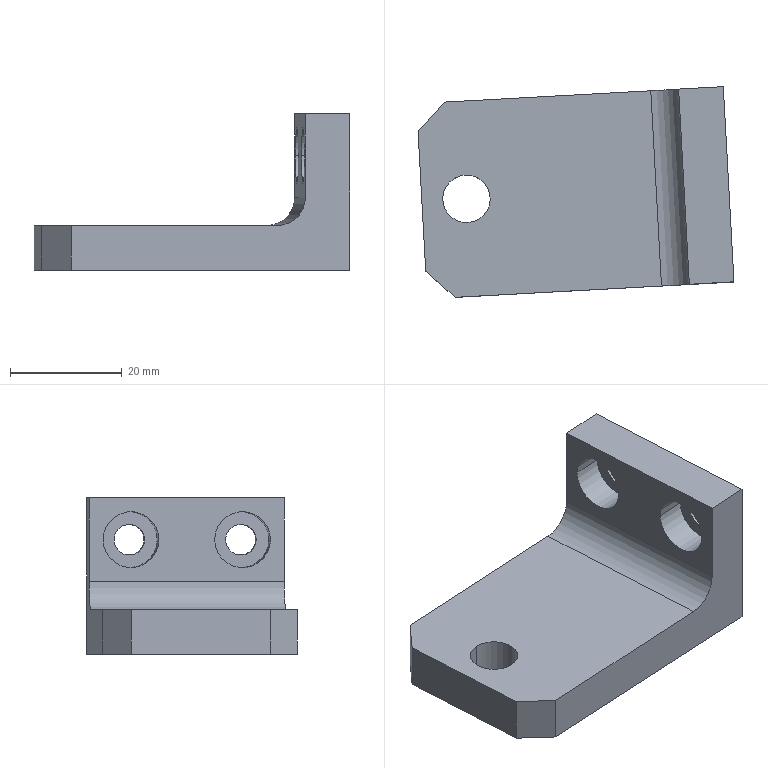Component | SolidWorks | BearingPressPartI-2 | 1 solid | 23 faces | box 56.56 x 37.68 x 28 mm | volume 19562 mm3 | plane 12 | cylinder 11 | commonest cylinder face diameters 10 x5 5.5 x4 8.5 x2
build123d program:
from build123d import *

# Parameters (mm, degrees)
BOSS_EXTRUDE1_DEPTH                             = 35
M5_HEX_SOCKET_HEAD_CAP_SCREW_CBORE1_D           = 5.5
M5_HEX_SOCKET_HEAD_CAP_SCREW_CBORE1_CBORE_D     = 10
M5_HEX_SOCKET_HEAD_CAP_SCREW_CBORE1_CBORE_DEPTH = 5.4
M10_TAPPED_HOLE1_D                              = 8.5
CHAMFER1_SIZE                                   = 5


with BuildPart() as part:
    # Sketch1 → Boss-Extrude1 (new body)
    with BuildSketch(Plane.XY):
        with BuildLine():
            Line((0, 0), (0, -55))
            Line((0, -55), (-28, -55))
            Line((-28, -55), (-28, -47))
            Line((-28, -47), (-13, -47))
            ThreePointArc((-13, -47), (-9.464, -45.536), (-8, -42))
            Line((-8, -42), (-8, 0))
            Line((-8, 0), (0, 0))
        make_face()
    extrude(amount=BOSS_EXTRUDE1_DEPTH)

    # M5 Hex Socket Head Cap Screw CBORE1 (through all)
    with Locations(Plane(origin=(0, -47, 0), x_dir=(-1, 0, 0), z_dir=(0, 1, 0))):
        with Locations((20.5, 7.5), (20.5, 27.5)):
            CounterBoreHole(M5_HEX_SOCKET_HEAD_CAP_SCREW_CBORE1_D / 2, M5_HEX_SOCKET_HEAD_CAP_SCREW_CBORE1_CBORE_D / 2, M5_HEX_SOCKET_HEAD_CAP_SCREW_CBORE1_CBORE_DEPTH)

    # M10 Tapped Hole1 (through all)
    with Locations(Plane.ZY.offset(8)):
        with Locations((17.5, -8)):
            Hole(M10_TAPPED_HOLE1_D / 2)

    # Chamfer1
    chamfer1_edges = [part.edges().sort_by_distance(p)[0] for p in [
        (-4, 0, 35),
        (-4, 0, 0),
    ]]
    chamfer(chamfer1_edges, length=CHAMFER1_SIZE)


solid = part.part

# Placed as in the assembly
solid = solid.moved(Location((341.568, 99.615, -284.318), (-90, -3.137, 90)))
STEP:
#1=COLOUR_RGB('',0.7922,0.8196,0.9333);
#2=FILL_AREA_STYLE_COLOUR('',#1);
#3=FILL_AREA_STYLE('',(#2));
#4=SURFACE_STYLE_FILL_AREA(#3);
#5=SURFACE_SIDE_STYLE('',(#4));
#6=SURFACE_STYLE_USAGE(.BOTH.,#5);
#7=PRESENTATION_STYLE_ASSIGNMENT((#6));
#8=CARTESIAN_POINT('',(13.734,4.46,-11.194));
#9=VERTEX_POINT('',#8);
#10=CARTESIAN_POINT('',(13.715,4.794,-11.194));
#11=VERTEX_POINT('',#10);
#12=CARTESIAN_POINT('',(13.724,4.627,-11.194));
#13=DIRECTION('',(0.,-0.,1.));
#14=DIRECTION('',(0.9985,0.05472,0.));
#15=AXIS2_PLACEMENT_3D('',#12,#13,#14);
#16=CIRCLE('',#15,0.1673);
#17=EDGE_CURVE('',#9,#11,#16,.T.);
#18=ORIENTED_EDGE('',*,*,#17,.F.);
#19=CARTESIAN_POINT('',(13.734,4.46,-10.879));
#20=VERTEX_POINT('',#19);
#21=CARTESIAN_POINT('',(13.734,4.46,-10.879));
#22=DIRECTION('',(0.,-0.,1.));
#23=VECTOR('',#22,39.37);
#24=LINE('',#21,#23);
#25=EDGE_CURVE('',#9,#20,#24,.T.);
#26=ORIENTED_EDGE('',*,*,#25,.T.);
#27=CARTESIAN_POINT('',(13.715,4.794,-10.879));
#28=VERTEX_POINT('',#27);
#29=CARTESIAN_POINT('',(13.724,4.627,-10.879));
#30=DIRECTION('',(0.,-0.,1.));
#31=DIRECTION('',(-0.05472,0.9985,0.));
#32=AXIS2_PLACEMENT_3D('',#29,#30,#31);
#33=CIRCLE('',#32,0.1673);
#34=EDGE_CURVE('',#20,#28,#33,.T.);
#35=ORIENTED_EDGE('',*,*,#34,.T.);
#36=CARTESIAN_POINT('',(13.715,4.794,-10.879));
#37=DIRECTION('',(0.,-0.,1.));
#38=VECTOR('',#37,39.37);
#39=LINE('',#36,#38);
#40=EDGE_CURVE('',#11,#28,#39,.T.);
#41=ORIENTED_EDGE('',*,*,#40,.F.);
#42=EDGE_LOOP('',(#18,#26,#35,#41));
#43=FACE_OUTER_BOUND('',#42,.T.);
#44=CARTESIAN_POINT('',(13.724,4.627,-10.879));
#45=DIRECTION('',(0.,-0.,1.));
#46=DIRECTION('',(-0.05472,0.9985,0.));
#47=AXIS2_PLACEMENT_3D('',#44,#45,#46);
#48=CYLINDRICAL_SURFACE('',#47,0.1673);
#49=ADVANCED_FACE('',(#43),#48,.F.);
#50=CARTESIAN_POINT('',(15.502,4.133,-10.387));
#51=VERTEX_POINT('',#50);
#52=CARTESIAN_POINT('',(15.481,4.526,-10.387));
#53=VERTEX_POINT('',#52);
#54=CARTESIAN_POINT('',(15.491,4.33,-10.387));
#55=DIRECTION('',(-0.9985,-0.05472,0.));
#56=DIRECTION('',(-0.05472,0.9985,0.));
#57=AXIS2_PLACEMENT_3D('',#54,#55,#56);
#58=CIRCLE('',#57,0.1969);
#59=EDGE_CURVE('',#51,#53,#58,.T.);
#60=ORIENTED_EDGE('',*,*,#59,.F.);
#61=CARTESIAN_POINT('',(15.29,4.121,-10.387));
#62=VERTEX_POINT('',#61);
#63=CARTESIAN_POINT('',(15.29,4.121,-10.387));
#64=DIRECTION('',(-0.9985,-0.05472,0.));
#65=VECTOR('',#64,39.37);
#66=LINE('',#63,#65);
#67=EDGE_CURVE('',#51,#62,#66,.T.);
#68=ORIENTED_EDGE('',*,*,#67,.T.);
#69=CARTESIAN_POINT('',(15.268,4.515,-10.387));
#70=VERTEX_POINT('',#69);
#71=CARTESIAN_POINT('',(15.279,4.318,-10.387));
#72=DIRECTION('',(-0.9985,-0.05472,0.));
#73=DIRECTION('',(-0.05472,0.9985,0.));
#74=AXIS2_PLACEMENT_3D('',#71,#72,#73);
#75=CIRCLE('',#74,0.1969);
#76=EDGE_CURVE('',#62,#70,#75,.T.);
#77=ORIENTED_EDGE('',*,*,#76,.T.);
#78=CARTESIAN_POINT('',(15.268,4.515,-10.387));
#79=DIRECTION('',(-0.9985,-0.05472,0.));
#80=VECTOR('',#79,39.37);
#81=LINE('',#78,#80);
#82=EDGE_CURVE('',#53,#70,#81,.T.);
#83=ORIENTED_EDGE('',*,*,#82,.F.);
#84=EDGE_LOOP('',(#60,#68,#77,#83));
#85=FACE_OUTER_BOUND('',#84,.T.);
#86=CARTESIAN_POINT('',(15.279,4.318,-10.387));
#87=DIRECTION('',(-0.9985,-0.05472,0.));
#88=DIRECTION('',(-0.05472,0.9985,0.));
#89=AXIS2_PLACEMENT_3D('',#86,#87,#88);
#90=CYLINDRICAL_SURFACE('',#89,0.1969);
#91=ADVANCED_FACE('',(#85),#90,.F.);
#92=CARTESIAN_POINT('',(15.599,4.227,-10.387));
#93=VERTEX_POINT('',#92);
#94=CARTESIAN_POINT('',(15.588,4.443,-10.387));
#95=VERTEX_POINT('',#94);
#96=CARTESIAN_POINT('',(15.594,4.335,-10.387));
#97=DIRECTION('',(-0.9985,-0.05472,0.));
#98=DIRECTION('',(0.,0.,1.));
#99=AXIS2_PLACEMENT_3D('',#96,#97,#98);
#100=CIRCLE('',#99,0.1083);
#101=EDGE_CURVE('',#93,#95,#100,.T.);
#102=ORIENTED_EDGE('',*,*,#101,.F.);
#103=CARTESIAN_POINT('',(15.497,4.221,-10.387));
#104=VERTEX_POINT('',#103);
#105=CARTESIAN_POINT('',(15.285,4.21,-10.387));
#106=DIRECTION('',(-0.9985,-0.05472,0.));
#107=VECTOR('',#106,39.37);
#108=LINE('',#105,#107);
#109=EDGE_CURVE('',#93,#104,#108,.T.);
#110=ORIENTED_EDGE('',*,*,#109,.T.);
#111=CARTESIAN_POINT('',(15.485,4.438,-10.387));
#112=VERTEX_POINT('',#111);
#113=CARTESIAN_POINT('',(15.491,4.33,-10.387));
#114=DIRECTION('',(-0.9985,-0.05472,0.));
#115=DIRECTION('',(-0.05472,0.9985,0.));
#116=AXIS2_PLACEMENT_3D('',#113,#114,#115);
#117=CIRCLE('',#116,0.1083);
#118=EDGE_CURVE('',#104,#112,#117,.T.);
#119=ORIENTED_EDGE('',*,*,#118,.T.);
#120=CARTESIAN_POINT('',(15.273,4.426,-10.387));
#121=DIRECTION('',(-0.9985,-0.05472,0.));
#122=VECTOR('',#121,39.37);
#123=LINE('',#120,#122);
#124=EDGE_CURVE('',#95,#112,#123,.T.);
#125=ORIENTED_EDGE('',*,*,#124,.F.);
#126=EDGE_LOOP('',(#102,#110,#119,#125));
#127=FACE_OUTER_BOUND('',#126,.T.);
#128=CARTESIAN_POINT('',(15.279,4.318,-10.387));
#129=DIRECTION('',(-0.9985,-0.05472,0.));
#130=DIRECTION('',(-0.05472,0.9985,0.));
#131=AXIS2_PLACEMENT_3D('',#128,#129,#130);
#132=CYLINDRICAL_SURFACE('',#131,0.1083);
#133=ADVANCED_FACE('',(#127),#132,.F.);
#134=CARTESIAN_POINT('',(15.459,4.919,-10.387));
#135=VERTEX_POINT('',#134);
#136=CARTESIAN_POINT('',(15.437,5.312,-10.387));
#137=VERTEX_POINT('',#136);
#138=CARTESIAN_POINT('',(15.448,5.116,-10.387));
#139=DIRECTION('',(-0.9985,-0.05472,0.));
#140=DIRECTION('',(-0.05472,0.9985,0.));
#141=AXIS2_PLACEMENT_3D('',#138,#139,#140);
#142=CIRCLE('',#141,0.1969);
#143=EDGE_CURVE('',#135,#137,#142,.T.);
#144=ORIENTED_EDGE('',*,*,#143,.F.);
#145=CARTESIAN_POINT('',(15.247,4.908,-10.387));
#146=VERTEX_POINT('',#145);
#147=CARTESIAN_POINT('',(15.247,4.908,-10.387));
#148=DIRECTION('',(-0.9985,-0.05472,0.));
#149=VECTOR('',#148,39.37);
#150=LINE('',#147,#149);
#151=EDGE_CURVE('',#135,#146,#150,.T.);
#152=ORIENTED_EDGE('',*,*,#151,.T.);
#153=CARTESIAN_POINT('',(15.225,5.301,-10.387));
#154=VERTEX_POINT('',#153);
#155=CARTESIAN_POINT('',(15.236,5.104,-10.387));
#156=DIRECTION('',(-0.9985,-0.05472,0.));
#157=DIRECTION('',(-0.05472,0.9985,0.));
#158=AXIS2_PLACEMENT_3D('',#155,#156,#157);
#159=CIRCLE('',#158,0.1969);
#160=EDGE_CURVE('',#146,#154,#159,.T.);
#161=ORIENTED_EDGE('',*,*,#160,.T.);
#162=CARTESIAN_POINT('',(15.225,5.301,-10.387));
#163=DIRECTION('',(-0.9985,-0.05472,0.));
#164=VECTOR('',#163,39.37);
#165=LINE('',#162,#164);
#166=EDGE_CURVE('',#137,#154,#165,.T.);
#167=ORIENTED_EDGE('',*,*,#166,.F.);
#168=EDGE_LOOP('',(#144,#152,#161,#167));
#169=FACE_OUTER_BOUND('',#168,.T.);
#170=CARTESIAN_POINT('',(15.236,5.104,-10.387));
#171=DIRECTION('',(-0.9985,-0.05472,0.));
#172=DIRECTION('',(-0.05472,0.9985,0.));
#173=AXIS2_PLACEMENT_3D('',#170,#171,#172);
#174=CYLINDRICAL_SURFACE('',#173,0.1969);
#175=ADVANCED_FACE('',(#169),#174,.F.);
#176=CARTESIAN_POINT('',(15.556,5.013,-10.387));
#177=VERTEX_POINT('',#176);
#178=CARTESIAN_POINT('',(15.545,5.23,-10.387));
#179=VERTEX_POINT('',#178);
#180=CARTESIAN_POINT('',(15.55,5.121,-10.387));
#181=DIRECTION('',(-0.9985,-0.05472,0.));
#182=DIRECTION('',(0.,0.,1.));
#183=AXIS2_PLACEMENT_3D('',#180,#181,#182);
#184=CIRCLE('',#183,0.1083);
#185=EDGE_CURVE('',#177,#179,#184,.T.);
#186=ORIENTED_EDGE('',*,*,#185,.F.);
#187=CARTESIAN_POINT('',(15.454,5.008,-10.387));
#188=VERTEX_POINT('',#187);
#189=CARTESIAN_POINT('',(15.242,4.996,-10.387));
#190=DIRECTION('',(-0.9985,-0.05472,0.));
#191=VECTOR('',#190,39.37);
#192=LINE('',#189,#191);
#193=EDGE_CURVE('',#177,#188,#192,.T.);
#194=ORIENTED_EDGE('',*,*,#193,.T.);
#195=CARTESIAN_POINT('',(15.442,5.224,-10.387));
#196=VERTEX_POINT('',#195);
#197=CARTESIAN_POINT('',(15.448,5.116,-10.387));
#198=DIRECTION('',(-0.9985,-0.05472,0.));
#199=DIRECTION('',(-0.05472,0.9985,0.));
#200=AXIS2_PLACEMENT_3D('',#197,#198,#199);
#201=CIRCLE('',#200,0.1083);
#202=EDGE_CURVE('',#188,#196,#201,.T.);
#203=ORIENTED_EDGE('',*,*,#202,.T.);
#204=CARTESIAN_POINT('',(15.23,5.212,-10.387));
#205=DIRECTION('',(-0.9985,-0.05472,0.));
#206=VECTOR('',#205,39.37);
#207=LINE('',#204,#206);
#208=EDGE_CURVE('',#179,#196,#207,.T.);
#209=ORIENTED_EDGE('',*,*,#208,.F.);
#210=EDGE_LOOP('',(#186,#194,#203,#209));
#211=FACE_OUTER_BOUND('',#210,.T.);
#212=CARTESIAN_POINT('',(15.236,5.104,-10.387));
#213=DIRECTION('',(-0.9985,-0.05472,0.));
#214=DIRECTION('',(-0.05472,0.9985,0.));
#215=AXIS2_PLACEMENT_3D('',#212,#213,#214);
#216=CYLINDRICAL_SURFACE('',#215,0.1083);
#217=ADVANCED_FACE('',(#211),#216,.F.);
#218=CARTESIAN_POINT('',(15.295,4.023,-10.682));
#219=VERTEX_POINT('',#218);
#220=CARTESIAN_POINT('',(15.295,4.023,-10.091));
#221=VERTEX_POINT('',#220);
#222=CARTESIAN_POINT('',(15.295,4.023,-10.091));
#223=DIRECTION('',(0.,-0.,1.));
#224=VECTOR('',#223,39.37);
#225=LINE('',#222,#224);
#226=EDGE_CURVE('',#219,#221,#225,.T.);
#227=ORIENTED_EDGE('',*,*,#226,.T.);
#228=CARTESIAN_POINT('',(15.22,5.399,-10.091));
#229=VERTEX_POINT('',#228);
#230=CARTESIAN_POINT('',(15.22,5.399,-10.091));
#231=DIRECTION('',(0.05472,-0.9985,-0.));
#232=VECTOR('',#231,39.37);
#233=LINE('',#230,#232);
#234=EDGE_CURVE('',#229,#221,#233,.T.);
#235=ORIENTED_EDGE('',*,*,#234,.F.);
#236=CARTESIAN_POINT('',(15.22,5.399,-10.682));
#237=VERTEX_POINT('',#236);
#238=CARTESIAN_POINT('',(15.22,5.399,-10.091));
#239=DIRECTION('',(0.,-0.,1.));
#240=VECTOR('',#239,39.37);
#241=LINE('',#238,#240);
#242=EDGE_CURVE('',#237,#229,#241,.T.);
#243=ORIENTED_EDGE('',*,*,#242,.F.);
#244=CARTESIAN_POINT('',(15.22,5.399,-10.682));
#245=DIRECTION('',(0.05472,-0.9985,-0.));
#246=VECTOR('',#245,39.37);
#247=LINE('',#244,#246);
#248=EDGE_CURVE('',#237,#219,#247,.T.);
#249=ORIENTED_EDGE('',*,*,#248,.T.);
#250=EDGE_LOOP('',(#227,#235,#243,#249));
#251=FACE_OUTER_BOUND('',#250,.T.);
#252=CARTESIAN_POINT('',(15.236,5.104,-10.387));
#253=DIRECTION('',(-0.9985,-0.05472,0.));
#254=DIRECTION('',(-0.05472,0.9985,0.));
#255=AXIS2_PLACEMENT_3D('',#252,#253,#254);
#256=CIRCLE('',#255,0.1969);
#257=EDGE_CURVE('',#154,#146,#256,.T.);
#258=ORIENTED_EDGE('',*,*,#257,.F.);
#259=ORIENTED_EDGE('',*,*,#160,.F.);
#260=EDGE_LOOP('',(#258,#259));
#261=FACE_BOUND('',#260,.T.);
#262=CARTESIAN_POINT('',(15.279,4.318,-10.387));
#263=DIRECTION('',(-0.9985,-0.05472,0.));
#264=DIRECTION('',(-0.05472,0.9985,0.));
#265=AXIS2_PLACEMENT_3D('',#262,#263,#264);
#266=CIRCLE('',#265,0.1969);
#267=EDGE_CURVE('',#70,#62,#266,.T.);
#268=ORIENTED_EDGE('',*,*,#267,.F.);
#269=ORIENTED_EDGE('',*,*,#76,.F.);
#270=EDGE_LOOP('',(#268,#269));
#271=FACE_BOUND('',#270,.T.);
#272=CARTESIAN_POINT('',(15.22,5.399,-10.091));
#273=DIRECTION('',(0.9985,0.05472,-0.));
#274=DIRECTION('',(0.05472,-0.9985,-0.));
#275=AXIS2_PLACEMENT_3D('',#272,#273,#274);
#276=PLANE('',#275);
#277=ADVANCED_FACE('',(#251,#261,#271),#276,.F.);
#278=CARTESIAN_POINT('',(13.383,5.101,-11.194));
#279=VERTEX_POINT('',#278);
#280=CARTESIAN_POINT('',(13.437,4.118,-11.194));
#281=VERTEX_POINT('',#280);
#282=CARTESIAN_POINT('',(13.372,5.298,-11.194));
#283=DIRECTION('',(0.05472,-0.9985,-0.));
#284=VECTOR('',#283,39.37);
#285=LINE('',#282,#284);
#286=EDGE_CURVE('',#279,#281,#285,.T.);
#287=ORIENTED_EDGE('',*,*,#286,.T.);
#288=CARTESIAN_POINT('',(13.437,4.118,-10.879));
#289=VERTEX_POINT('',#288);
#290=CARTESIAN_POINT('',(13.437,4.118,-10.879));
#291=DIRECTION('',(0.,-0.,1.));
#292=VECTOR('',#291,39.37);
#293=LINE('',#290,#292);
#294=EDGE_CURVE('',#281,#289,#293,.T.);
#295=ORIENTED_EDGE('',*,*,#294,.T.);
#296=CARTESIAN_POINT('',(13.383,5.101,-10.879));
#297=VERTEX_POINT('',#296);
#298=CARTESIAN_POINT('',(13.372,5.298,-10.879));
#299=DIRECTION('',(0.05472,-0.9985,-0.));
#300=VECTOR('',#299,39.37);
#301=LINE('',#298,#300);
#302=EDGE_CURVE('',#297,#289,#301,.T.);
#303=ORIENTED_EDGE('',*,*,#302,.F.);
#304=CARTESIAN_POINT('',(13.383,5.101,-10.879));
#305=DIRECTION('',(-0.,0.,-1.));
#306=VECTOR('',#305,39.37);
#307=LINE('',#304,#306);
#308=EDGE_CURVE('',#297,#279,#307,.T.);
#309=ORIENTED_EDGE('',*,*,#308,.T.);
#310=EDGE_LOOP('',(#287,#295,#303,#309));
#311=FACE_OUTER_BOUND('',#310,.T.);
#312=CARTESIAN_POINT('',(13.372,5.298,-10.879));
#313=DIRECTION('',(0.9985,0.05472,-0.));
#314=DIRECTION('',(0.05472,-0.9985,-0.));
#315=AXIS2_PLACEMENT_3D('',#312,#313,#314);
#316=PLANE('',#315);
#317=ADVANCED_FACE('',(#311),#316,.F.);
#318=CARTESIAN_POINT('',(13.724,4.627,-10.879));
#319=DIRECTION('',(0.,-0.,1.));
#320=DIRECTION('',(-0.05472,0.9985,0.));
#321=AXIS2_PLACEMENT_3D('',#318,#319,#320);
#322=CIRCLE('',#321,0.1673);
#323=EDGE_CURVE('',#28,#20,#322,.T.);
#324=ORIENTED_EDGE('',*,*,#323,.F.);
#325=ORIENTED_EDGE('',*,*,#34,.F.);
#326=EDGE_LOOP('',(#324,#325));
#327=FACE_BOUND('',#326,.T.);
#328=ORIENTED_EDGE('',*,*,#302,.T.);
#329=CARTESIAN_POINT('',(13.644,3.933,-10.879));
#330=VERTEX_POINT('',#329);
#331=CARTESIAN_POINT('',(13.437,4.118,-10.879));
#332=DIRECTION('',(0.7447,-0.6674,-0.));
#333=VECTOR('',#332,39.37);
#334=LINE('',#331,#333);
#335=EDGE_CURVE('',#289,#330,#334,.T.);
#336=ORIENTED_EDGE('',*,*,#335,.T.);
#337=CARTESIAN_POINT('',(15.099,4.012,-10.879));
#338=VERTEX_POINT('',#337);
#339=CARTESIAN_POINT('',(15.099,4.012,-10.879));
#340=DIRECTION('',(0.9985,0.05472,-0.));
#341=VECTOR('',#340,39.37);
#342=LINE('',#339,#341);
#343=EDGE_CURVE('',#330,#338,#342,.T.);
#344=ORIENTED_EDGE('',*,*,#343,.T.);
#345=CARTESIAN_POINT('',(15.023,5.388,-10.879));
#346=VERTEX_POINT('',#345);
#347=CARTESIAN_POINT('',(15.023,5.388,-10.879));
#348=DIRECTION('',(0.05472,-0.9985,-0.));
#349=VECTOR('',#348,39.37);
#350=LINE('',#347,#349);
#351=EDGE_CURVE('',#346,#338,#350,.T.);
#352=ORIENTED_EDGE('',*,*,#351,.F.);
#353=CARTESIAN_POINT('',(13.569,5.309,-10.879));
#354=VERTEX_POINT('',#353);
#355=CARTESIAN_POINT('',(15.023,5.388,-10.879));
#356=DIRECTION('',(0.9985,0.05472,-0.));
#357=VECTOR('',#356,39.37);
#358=LINE('',#355,#357);
#359=EDGE_CURVE('',#354,#346,#358,.T.);
#360=ORIENTED_EDGE('',*,*,#359,.F.);
#361=CARTESIAN_POINT('',(13.569,5.309,-10.879));
#362=DIRECTION('',(-0.6674,-0.7447,-0.));
#363=VECTOR('',#362,39.37);
#364=LINE('',#361,#363);
#365=EDGE_CURVE('',#354,#297,#364,.T.);
#366=ORIENTED_EDGE('',*,*,#365,.T.);
#367=EDGE_LOOP('',(#328,#336,#344,#352,#360,#366));
#368=FACE_OUTER_BOUND('',#367,.T.);
#369=CARTESIAN_POINT('',(15.023,5.388,-10.879));
#370=DIRECTION('',(-0.,0.,-1.));
#371=DIRECTION('',(0.05472,-0.9985,-0.));
#372=AXIS2_PLACEMENT_3D('',#369,#370,#371);
#373=PLANE('',#372);
#374=ADVANCED_FACE('',(#327,#368),#373,.F.);
#375=CARTESIAN_POINT('',(15.099,4.012,-10.682));
#376=DIRECTION('',(0.05472,-0.9985,-0.));
#377=DIRECTION('',(0.,0.,1.));
#378=AXIS2_PLACEMENT_3D('',#375,#376,#377);
#379=CIRCLE('',#378,0.1969);
#380=EDGE_CURVE('',#338,#219,#379,.T.);
#381=ORIENTED_EDGE('',*,*,#380,.T.);
#382=ORIENTED_EDGE('',*,*,#248,.F.);
#383=CARTESIAN_POINT('',(15.023,5.388,-10.682));
#384=DIRECTION('',(0.05472,-0.9985,-0.));
#385=DIRECTION('',(0.,0.,1.));
#386=AXIS2_PLACEMENT_3D('',#383,#384,#385);
#387=CIRCLE('',#386,0.1969);
#388=EDGE_CURVE('',#346,#237,#387,.T.);
#389=ORIENTED_EDGE('',*,*,#388,.F.);
#390=ORIENTED_EDGE('',*,*,#351,.T.);
#391=EDGE_LOOP('',(#381,#382,#389,#390));
#392=FACE_OUTER_BOUND('',#391,.T.);
#393=CARTESIAN_POINT('',(15.023,5.388,-10.682));
#394=DIRECTION('',(0.05472,-0.9985,-0.));
#395=DIRECTION('',(0.,0.,1.));
#396=AXIS2_PLACEMENT_3D('',#393,#394,#395);
#397=CYLINDRICAL_SURFACE('',#396,0.1969);
#398=ADVANCED_FACE('',(#392),#397,.F.);
#399=CARTESIAN_POINT('',(15.61,4.04,-10.091));
#400=VERTEX_POINT('',#399);
#401=CARTESIAN_POINT('',(15.61,4.04,-10.091));
#402=DIRECTION('',(0.9985,0.05472,-0.));
#403=VECTOR('',#402,39.37);
#404=LINE('',#401,#403);
#405=EDGE_CURVE('',#221,#400,#404,.T.);
#406=ORIENTED_EDGE('',*,*,#405,.T.);
#407=CARTESIAN_POINT('',(15.534,5.416,-10.091));
#408=VERTEX_POINT('',#407);
#409=CARTESIAN_POINT('',(15.534,5.416,-10.091));
#410=DIRECTION('',(0.05472,-0.9985,-0.));
#411=VECTOR('',#410,39.37);
#412=LINE('',#409,#411);
#413=EDGE_CURVE('',#408,#400,#412,.T.);
#414=ORIENTED_EDGE('',*,*,#413,.F.);
#415=CARTESIAN_POINT('',(15.534,5.416,-10.091));
#416=DIRECTION('',(0.9985,0.05472,-0.));
#417=VECTOR('',#416,39.37);
#418=LINE('',#415,#417);
#419=EDGE_CURVE('',#229,#408,#418,.T.);
#420=ORIENTED_EDGE('',*,*,#419,.F.);
#421=ORIENTED_EDGE('',*,*,#234,.T.);
#422=EDGE_LOOP('',(#406,#414,#420,#421));
#423=FACE_OUTER_BOUND('',#422,.T.);
#424=CARTESIAN_POINT('',(15.534,5.416,-10.091));
#425=DIRECTION('',(-0.,0.,-1.));
#426=DIRECTION('',(0.05472,-0.9985,-0.));
#427=AXIS2_PLACEMENT_3D('',#424,#425,#426);
#428=PLANE('',#427);
#429=ADVANCED_FACE('',(#423),#428,.F.);
#430=CARTESIAN_POINT('',(15.594,4.335,-10.387));
#431=DIRECTION('',(-0.9985,-0.05472,0.));
#432=DIRECTION('',(0.,0.,1.));
#433=AXIS2_PLACEMENT_3D('',#430,#431,#432);
#434=CIRCLE('',#433,0.1083);
#435=EDGE_CURVE('',#95,#93,#434,.T.);
#436=ORIENTED_EDGE('',*,*,#435,.T.);
#437=ORIENTED_EDGE('',*,*,#101,.T.);
#438=EDGE_LOOP('',(#436,#437));
#439=FACE_BOUND('',#438,.T.);
#440=CARTESIAN_POINT('',(15.55,5.121,-10.387));
#441=DIRECTION('',(-0.9985,-0.05472,0.));
#442=DIRECTION('',(0.,0.,1.));
#443=AXIS2_PLACEMENT_3D('',#440,#441,#442);
#444=CIRCLE('',#443,0.1083);
#445=EDGE_CURVE('',#179,#177,#444,.T.);
#446=ORIENTED_EDGE('',*,*,#445,.T.);
#447=ORIENTED_EDGE('',*,*,#185,.T.);
#448=EDGE_LOOP('',(#446,#447));
#449=FACE_BOUND('',#448,.T.);
#450=CARTESIAN_POINT('',(15.61,4.04,-11.194));
#451=VERTEX_POINT('',#450);
#452=CARTESIAN_POINT('',(15.61,4.04,-11.194));
#453=DIRECTION('',(-0.,0.,-1.));
#454=VECTOR('',#453,39.37);
#455=LINE('',#452,#454);
#456=EDGE_CURVE('',#400,#451,#455,.T.);
#457=ORIENTED_EDGE('',*,*,#456,.T.);
#458=CARTESIAN_POINT('',(15.534,5.416,-11.194));
#459=VERTEX_POINT('',#458);
#460=CARTESIAN_POINT('',(15.534,5.416,-11.194));
#461=DIRECTION('',(0.05472,-0.9985,-0.));
#462=VECTOR('',#461,39.37);
#463=LINE('',#460,#462);
#464=EDGE_CURVE('',#459,#451,#463,.T.);
#465=ORIENTED_EDGE('',*,*,#464,.F.);
#466=CARTESIAN_POINT('',(15.534,5.416,-11.194));
#467=DIRECTION('',(-0.,0.,-1.));
#468=VECTOR('',#467,39.37);
#469=LINE('',#466,#468);
#470=EDGE_CURVE('',#408,#459,#469,.T.);
#471=ORIENTED_EDGE('',*,*,#470,.F.);
#472=ORIENTED_EDGE('',*,*,#413,.T.);
#473=EDGE_LOOP('',(#457,#465,#471,#472));
#474=FACE_OUTER_BOUND('',#473,.T.);
#475=CARTESIAN_POINT('',(15.534,5.416,-11.194));
#476=DIRECTION('',(-0.9985,-0.05472,0.));
#477=DIRECTION('',(0.,-0.,1.));
#478=AXIS2_PLACEMENT_3D('',#475,#476,#477);
#479=PLANE('',#478);
#480=ADVANCED_FACE('',(#439,#449,#474),#479,.F.);
#481=CARTESIAN_POINT('',(13.724,4.627,-11.194));
#482=DIRECTION('',(0.,-0.,1.));
#483=DIRECTION('',(0.9985,0.05472,0.));
#484=AXIS2_PLACEMENT_3D('',#481,#482,#483);
#485=CIRCLE('',#484,0.1673);
#486=EDGE_CURVE('',#11,#9,#485,.T.);
#487=ORIENTED_EDGE('',*,*,#486,.T.);
#488=ORIENTED_EDGE('',*,*,#17,.T.);
#489=EDGE_LOOP('',(#487,#488));
#490=FACE_BOUND('',#489,.T.);
#491=CARTESIAN_POINT('',(13.644,3.933,-11.194));
#492=VERTEX_POINT('',#491);
#493=CARTESIAN_POINT('',(13.448,3.922,-11.194));
#494=DIRECTION('',(-0.9985,-0.05472,0.));
#495=VECTOR('',#494,39.37);
#496=LINE('',#493,#495);
#497=EDGE_CURVE('',#451,#492,#496,.T.);
#498=ORIENTED_EDGE('',*,*,#497,.T.);
#499=CARTESIAN_POINT('',(13.437,4.118,-11.194));
#500=DIRECTION('',(-0.7447,0.6674,0.));
#501=VECTOR('',#500,39.37);
#502=LINE('',#499,#501);
#503=EDGE_CURVE('',#492,#281,#502,.T.);
#504=ORIENTED_EDGE('',*,*,#503,.T.);
#505=ORIENTED_EDGE('',*,*,#286,.F.);
#506=CARTESIAN_POINT('',(13.569,5.309,-11.194));
#507=VERTEX_POINT('',#506);
#508=CARTESIAN_POINT('',(13.569,5.309,-11.194));
#509=DIRECTION('',(0.6674,0.7447,-0.));
#510=VECTOR('',#509,39.37);
#511=LINE('',#508,#510);
#512=EDGE_CURVE('',#279,#507,#511,.T.);
#513=ORIENTED_EDGE('',*,*,#512,.T.);
#514=CARTESIAN_POINT('',(13.372,5.298,-11.194));
#515=DIRECTION('',(-0.9985,-0.05472,0.));
#516=VECTOR('',#515,39.37);
#517=LINE('',#514,#516);
#518=EDGE_CURVE('',#459,#507,#517,.T.);
#519=ORIENTED_EDGE('',*,*,#518,.F.);
#520=ORIENTED_EDGE('',*,*,#464,.T.);
#521=EDGE_LOOP('',(#498,#504,#505,#513,#519,#520));
#522=FACE_OUTER_BOUND('',#521,.T.);
#523=CARTESIAN_POINT('',(13.372,5.298,-11.194));
#524=DIRECTION('',(0.,-0.,1.));
#525=DIRECTION('',(0.9985,0.05472,-0.));
#526=AXIS2_PLACEMENT_3D('',#523,#524,#525);
#527=PLANE('',#526);
#528=ADVANCED_FACE('',(#490,#522),#527,.F.);
#529=ORIENTED_EDGE('',*,*,#518,.T.);
#530=CARTESIAN_POINT('',(13.569,5.309,-10.682));
#531=DIRECTION('',(0.,-0.,1.));
#532=VECTOR('',#531,39.37);
#533=LINE('',#530,#532);
#534=EDGE_CURVE('',#507,#354,#533,.T.);
#535=ORIENTED_EDGE('',*,*,#534,.T.);
#536=ORIENTED_EDGE('',*,*,#359,.T.);
#537=ORIENTED_EDGE('',*,*,#388,.T.);
#538=ORIENTED_EDGE('',*,*,#242,.T.);
#539=ORIENTED_EDGE('',*,*,#419,.T.);
#540=ORIENTED_EDGE('',*,*,#470,.T.);
#541=EDGE_LOOP('',(#529,#535,#536,#537,#538,#539,#540));
#542=FACE_OUTER_BOUND('',#541,.T.);
#543=CARTESIAN_POINT('',(15.023,5.388,-10.682));
#544=DIRECTION('',(0.05472,-0.9985,-0.));
#545=DIRECTION('',(0.,-0.,1.));
#546=AXIS2_PLACEMENT_3D('',#543,#544,#545);
#547=PLANE('',#546);
#548=ADVANCED_FACE('',(#542),#547,.F.);
#549=ORIENTED_EDGE('',*,*,#343,.F.);
#550=CARTESIAN_POINT('',(13.644,3.933,-11.194));
#551=DIRECTION('',(-0.,0.,-1.));
#552=VECTOR('',#551,39.37);
#553=LINE('',#550,#552);
#554=EDGE_CURVE('',#330,#492,#553,.T.);
#555=ORIENTED_EDGE('',*,*,#554,.T.);
#556=ORIENTED_EDGE('',*,*,#497,.F.);
#557=ORIENTED_EDGE('',*,*,#456,.F.);
#558=ORIENTED_EDGE('',*,*,#405,.F.);
#559=ORIENTED_EDGE('',*,*,#226,.F.);
#560=ORIENTED_EDGE('',*,*,#380,.F.);
#561=EDGE_LOOP('',(#549,#555,#556,#557,#558,#559,#560));
#562=FACE_OUTER_BOUND('',#561,.T.);
#563=CARTESIAN_POINT('',(15.099,4.012,-10.682));
#564=DIRECTION('',(0.05472,-0.9985,-0.));
#565=DIRECTION('',(0.,-0.,1.));
#566=AXIS2_PLACEMENT_3D('',#563,#564,#565);
#567=PLANE('',#566);
#568=ADVANCED_FACE('',(#562),#567,.T.);
#569=ORIENTED_EDGE('',*,*,#193,.F.);
#570=ORIENTED_EDGE('',*,*,#445,.F.);
#571=ORIENTED_EDGE('',*,*,#208,.T.);
#572=CARTESIAN_POINT('',(15.448,5.116,-10.387));
#573=DIRECTION('',(-0.9985,-0.05472,0.));
#574=DIRECTION('',(-0.05472,0.9985,0.));
#575=AXIS2_PLACEMENT_3D('',#572,#573,#574);
#576=CIRCLE('',#575,0.1083);
#577=EDGE_CURVE('',#196,#188,#576,.T.);
#578=ORIENTED_EDGE('',*,*,#577,.T.);
#579=EDGE_LOOP('',(#569,#570,#571,#578));
#580=FACE_OUTER_BOUND('',#579,.T.);
#581=CARTESIAN_POINT('',(15.236,5.104,-10.387));
#582=DIRECTION('',(-0.9985,-0.05472,0.));
#583=DIRECTION('',(-0.05472,0.9985,0.));
#584=AXIS2_PLACEMENT_3D('',#581,#582,#583);
#585=CYLINDRICAL_SURFACE('',#584,0.1083);
#586=ADVANCED_FACE('',(#580),#585,.F.);
#587=ORIENTED_EDGE('',*,*,#577,.F.);
#588=ORIENTED_EDGE('',*,*,#202,.F.);
#589=EDGE_LOOP('',(#587,#588));
#590=FACE_BOUND('',#589,.T.);
#591=CARTESIAN_POINT('',(15.448,5.116,-10.387));
#592=DIRECTION('',(-0.9985,-0.05472,0.));
#593=DIRECTION('',(-0.05472,0.9985,0.));
#594=AXIS2_PLACEMENT_3D('',#591,#592,#593);
#595=CIRCLE('',#594,0.1969);
#596=EDGE_CURVE('',#137,#135,#595,.T.);
#597=ORIENTED_EDGE('',*,*,#596,.T.);
#598=ORIENTED_EDGE('',*,*,#143,.T.);
#599=EDGE_LOOP('',(#597,#598));
#600=FACE_OUTER_BOUND('',#599,.T.);
#601=CARTESIAN_POINT('',(15.448,5.116,-10.495));
#602=DIRECTION('',(0.9985,0.05472,-0.));
#603=DIRECTION('',(0.05472,-0.9985,-0.));
#604=AXIS2_PLACEMENT_3D('',#601,#602,#603);
#605=PLANE('',#604);
#606=ADVANCED_FACE('',(#590,#600),#605,.F.);
#607=ORIENTED_EDGE('',*,*,#151,.F.);
#608=ORIENTED_EDGE('',*,*,#596,.F.);
#609=ORIENTED_EDGE('',*,*,#166,.T.);
#610=ORIENTED_EDGE('',*,*,#257,.T.);
#611=EDGE_LOOP('',(#607,#608,#609,#610));
#612=FACE_OUTER_BOUND('',#611,.T.);
#613=CARTESIAN_POINT('',(15.236,5.104,-10.387));
#614=DIRECTION('',(-0.9985,-0.05472,0.));
#615=DIRECTION('',(-0.05472,0.9985,0.));
#616=AXIS2_PLACEMENT_3D('',#613,#614,#615);
#617=CYLINDRICAL_SURFACE('',#616,0.1969);
#618=ADVANCED_FACE('',(#612),#617,.F.);
#619=ORIENTED_EDGE('',*,*,#109,.F.);
#620=ORIENTED_EDGE('',*,*,#435,.F.);
#621=ORIENTED_EDGE('',*,*,#124,.T.);
#622=CARTESIAN_POINT('',(15.491,4.33,-10.387));
#623=DIRECTION('',(-0.9985,-0.05472,0.));
#624=DIRECTION('',(-0.05472,0.9985,0.));
#625=AXIS2_PLACEMENT_3D('',#622,#623,#624);
#626=CIRCLE('',#625,0.1083);
#627=EDGE_CURVE('',#112,#104,#626,.T.);
#628=ORIENTED_EDGE('',*,*,#627,.T.);
#629=EDGE_LOOP('',(#619,#620,#621,#628));
#630=FACE_OUTER_BOUND('',#629,.T.);
#631=CARTESIAN_POINT('',(15.279,4.318,-10.387));
#632=DIRECTION('',(-0.9985,-0.05472,0.));
#633=DIRECTION('',(-0.05472,0.9985,0.));
#634=AXIS2_PLACEMENT_3D('',#631,#632,#633);
#635=CYLINDRICAL_SURFACE('',#634,0.1083);
#636=ADVANCED_FACE('',(#630),#635,.F.);
#637=ORIENTED_EDGE('',*,*,#627,.F.);
#638=ORIENTED_EDGE('',*,*,#118,.F.);
#639=EDGE_LOOP('',(#637,#638));
#640=FACE_BOUND('',#639,.T.);
#641=CARTESIAN_POINT('',(15.491,4.33,-10.387));
#642=DIRECTION('',(-0.9985,-0.05472,0.));
#643=DIRECTION('',(-0.05472,0.9985,0.));
#644=AXIS2_PLACEMENT_3D('',#641,#642,#643);
#645=CIRCLE('',#644,0.1969);
#646=EDGE_CURVE('',#53,#51,#645,.T.);
#647=ORIENTED_EDGE('',*,*,#646,.T.);
#648=ORIENTED_EDGE('',*,*,#59,.T.);
#649=EDGE_LOOP('',(#647,#648));
#650=FACE_OUTER_BOUND('',#649,.T.);
#651=CARTESIAN_POINT('',(15.491,4.33,-10.495));
#652=DIRECTION('',(0.9985,0.05472,-0.));
#653=DIRECTION('',(0.05472,-0.9985,-0.));
#654=AXIS2_PLACEMENT_3D('',#651,#652,#653);
#655=PLANE('',#654);
#656=ADVANCED_FACE('',(#640,#650),#655,.F.);
#657=ORIENTED_EDGE('',*,*,#67,.F.);
#658=ORIENTED_EDGE('',*,*,#646,.F.);
#659=ORIENTED_EDGE('',*,*,#82,.T.);
#660=ORIENTED_EDGE('',*,*,#267,.T.);
#661=EDGE_LOOP('',(#657,#658,#659,#660));
#662=FACE_OUTER_BOUND('',#661,.T.);
#663=CARTESIAN_POINT('',(15.279,4.318,-10.387));
#664=DIRECTION('',(-0.9985,-0.05472,0.));
#665=DIRECTION('',(-0.05472,0.9985,0.));
#666=AXIS2_PLACEMENT_3D('',#663,#664,#665);
#667=CYLINDRICAL_SURFACE('',#666,0.1969);
#668=ADVANCED_FACE('',(#662),#667,.F.);
#669=ORIENTED_EDGE('',*,*,#25,.F.);
#670=ORIENTED_EDGE('',*,*,#486,.F.);
#671=ORIENTED_EDGE('',*,*,#40,.T.);
#672=ORIENTED_EDGE('',*,*,#323,.T.);
#673=EDGE_LOOP('',(#669,#670,#671,#672));
#674=FACE_OUTER_BOUND('',#673,.T.);
#675=CARTESIAN_POINT('',(13.724,4.627,-10.879));
#676=DIRECTION('',(0.,-0.,1.));
#677=DIRECTION('',(-0.05472,0.9985,0.));
#678=AXIS2_PLACEMENT_3D('',#675,#676,#677);
#679=CYLINDRICAL_SURFACE('',#678,0.1673);
#680=ADVANCED_FACE('',(#674),#679,.F.);
#681=ORIENTED_EDGE('',*,*,#503,.F.);
#682=ORIENTED_EDGE('',*,*,#554,.F.);
#683=ORIENTED_EDGE('',*,*,#335,.F.);
#684=ORIENTED_EDGE('',*,*,#294,.F.);
#685=EDGE_LOOP('',(#681,#682,#683,#684));
#686=FACE_OUTER_BOUND('',#685,.T.);
#687=CARTESIAN_POINT('',(13.437,4.118,-10.879));
#688=DIRECTION('',(-0.6674,-0.7447,-0.));
#689=DIRECTION('',(-0.,0.,-1.));
#690=AXIS2_PLACEMENT_3D('',#687,#688,#689);
#691=PLANE('',#690);
#692=ADVANCED_FACE('',(#686),#691,.T.);
#693=ORIENTED_EDGE('',*,*,#512,.F.);
#694=ORIENTED_EDGE('',*,*,#308,.F.);
#695=ORIENTED_EDGE('',*,*,#365,.F.);
#696=ORIENTED_EDGE('',*,*,#534,.F.);
#697=EDGE_LOOP('',(#693,#694,#695,#696));
#698=FACE_OUTER_BOUND('',#697,.T.);
#699=CARTESIAN_POINT('',(13.569,5.309,-10.682));
#700=DIRECTION('',(0.7447,-0.6674,-0.));
#701=DIRECTION('',(0.,-0.,1.));
#702=AXIS2_PLACEMENT_3D('',#699,#700,#701);
#703=PLANE('',#702);
#704=ADVANCED_FACE('',(#698),#703,.F.);
#705=CLOSED_SHELL('',(#49,#91,#133,#175,#217,#277,#317,#374,#398,#429,#480,#528,#548,#568,#586,#606,#618,#636,#656,#668,#680,#692,#704));
#706=MANIFOLD_SOLID_BREP('',#705);
#707=STYLED_ITEM('',(#7),#706);
#708=PRESENTATION_LAYER_ASSIGNMENT('','',(#707));
#709=(LENGTH_UNIT()NAMED_UNIT(*)SI_UNIT($,.METRE.));
#710=LENGTH_MEASURE_WITH_UNIT(LENGTH_MEASURE(0.0254),#709);
#711=DIMENSIONAL_EXPONENTS(1.,0.,0.,0.,0.,0.,0.);
#712=(CONVERSION_BASED_UNIT('',#710)LENGTH_UNIT()NAMED_UNIT(#711));
#713=UNCERTAINTY_MEASURE_WITH_UNIT(LENGTH_MEASURE(0.00001),#712,'','');
#714=(NAMED_UNIT(*)PLANE_ANGLE_UNIT()SI_UNIT($,.RADIAN.));
#715=(NAMED_UNIT(*)SI_UNIT($,.STERADIAN.)SOLID_ANGLE_UNIT());
#716=(GEOMETRIC_REPRESENTATION_CONTEXT(3)GLOBAL_UNCERTAINTY_ASSIGNED_CONTEXT((#713))GLOBAL_UNIT_ASSIGNED_CONTEXT((#712,#714,#715))REPRESENTATION_CONTEXT('',''));
#717=MECHANICAL_DESIGN_GEOMETRIC_PRESENTATION_REPRESENTATION('',(#707),#716);
#718=CARTESIAN_POINT('',(0.,0.,0.));
#719=DIRECTION('',(0.,0.,1.));
#720=DIRECTION('',(1.,0.,0.));
#721=AXIS2_PLACEMENT_3D('',#718,#719,#720);
#722=(LENGTH_UNIT()NAMED_UNIT(*)SI_UNIT($,.METRE.));
#723=LENGTH_MEASURE_WITH_UNIT(LENGTH_MEASURE(0.0254),#722);
#724=DIMENSIONAL_EXPONENTS(1.,0.,0.,0.,0.,0.,0.);
#725=(CONVERSION_BASED_UNIT('',#723)LENGTH_UNIT()NAMED_UNIT(#724));
#726=UNCERTAINTY_MEASURE_WITH_UNIT(LENGTH_MEASURE(0.00001),#725,'','');
#727=(NAMED_UNIT(*)PLANE_ANGLE_UNIT()SI_UNIT($,.RADIAN.));
#728=(NAMED_UNIT(*)SI_UNIT($,.STERADIAN.)SOLID_ANGLE_UNIT());
#729=(GEOMETRIC_REPRESENTATION_CONTEXT(3)GLOBAL_UNCERTAINTY_ASSIGNED_CONTEXT((#726))GLOBAL_UNIT_ASSIGNED_CONTEXT((#725,#727,#728))REPRESENTATION_CONTEXT('',''));
#730=ADVANCED_BREP_SHAPE_REPRESENTATION('',(#706,#721),#729);